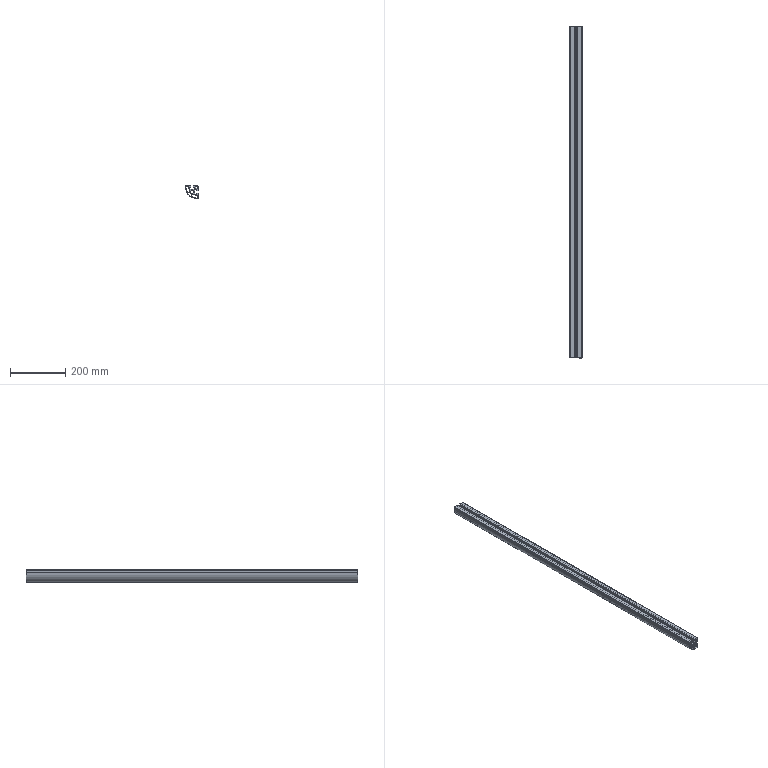Component | SolidWorks | 40-40AluminumProfileFrame-1_NFSR8-4545-100AA-2-2 | 1 solid | 97 faces | volume 873077 mm3 | plane 56 | cylinder 41 | commonest cylinder face diameters 4 x11 2 x11 1 x4 10.5 x3 1.46 x3 66 x3 16.5 x3 70 x1